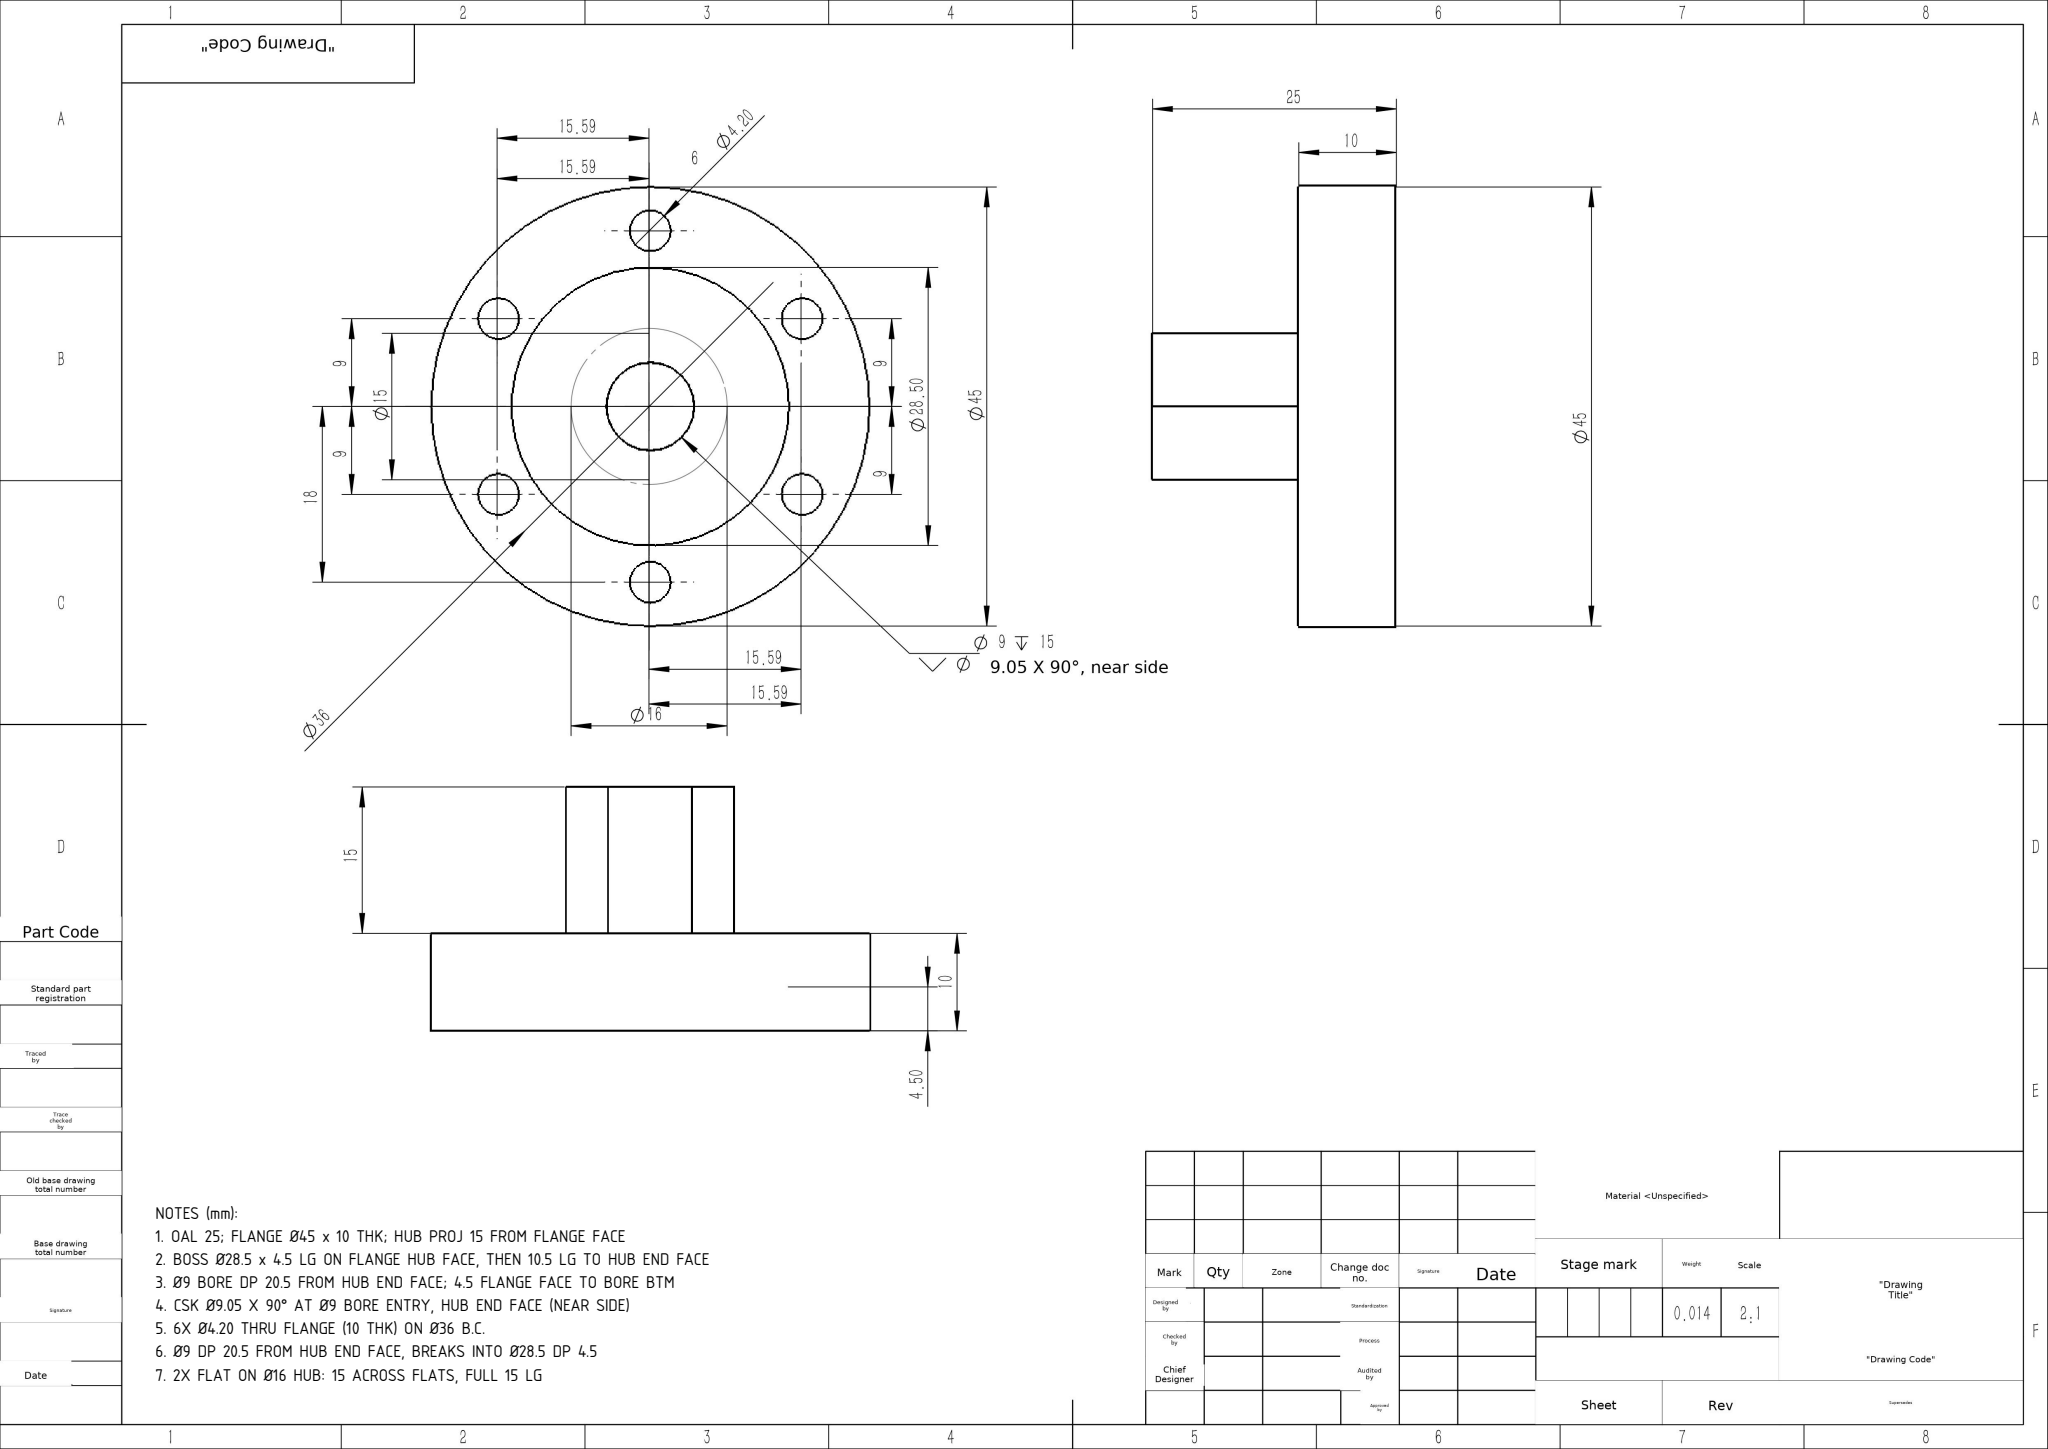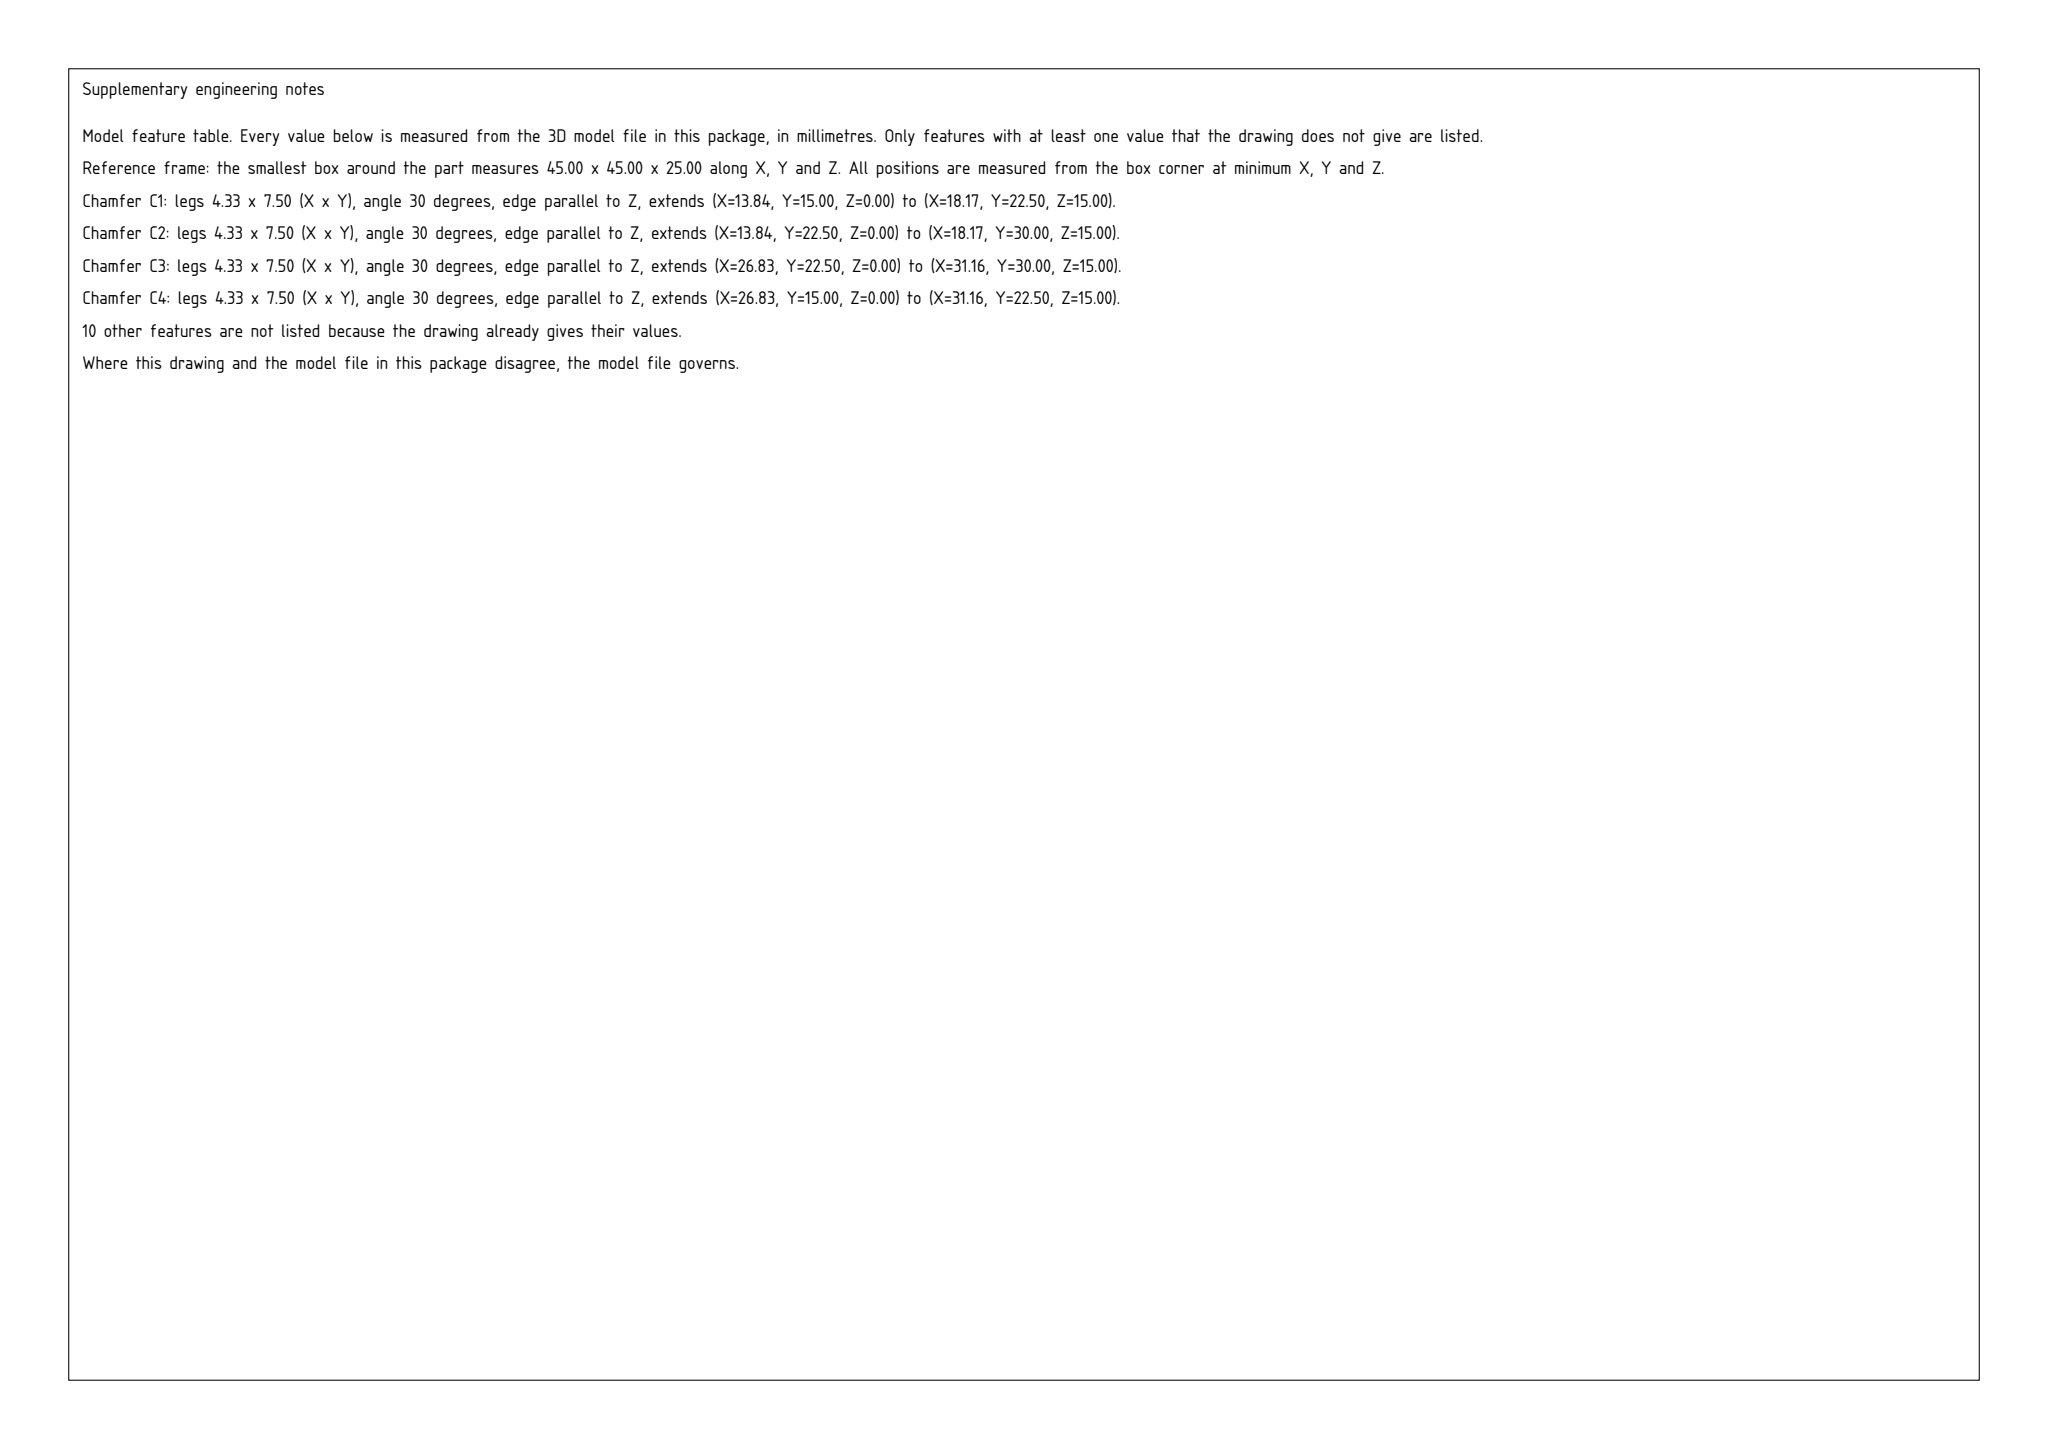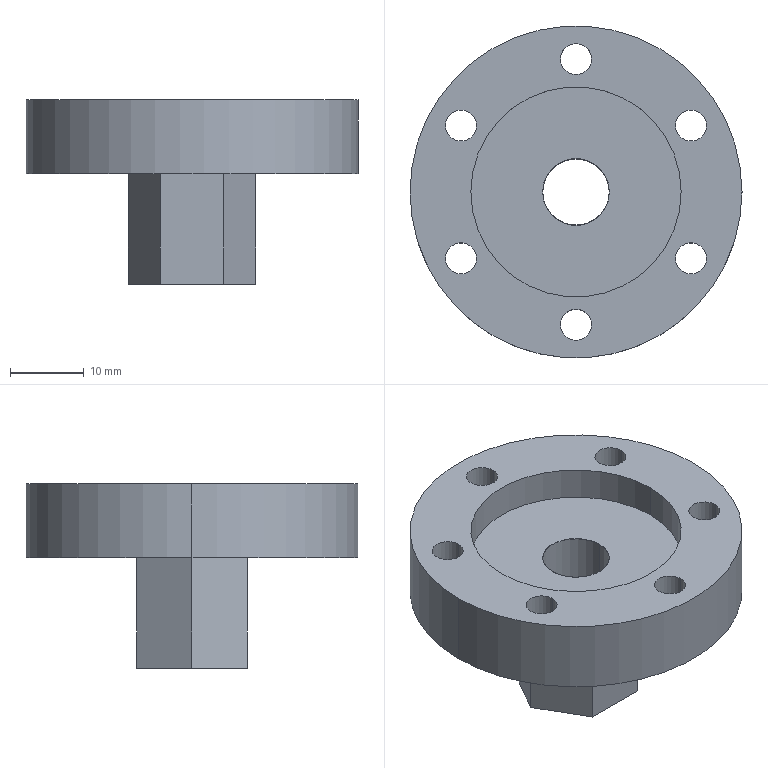Part | SolidWorks | mm | 1 solid | 30 faces | box 45 x 45 x 25 mm | volume 13821 mm3 | cylinder 18 | plane 10 | cone 2 | commonest cylinder face diameters 4.2 x12 9 x2 28.5 x2 45 x2
Drawing notes:
OAL 25; FLANGE Ø45 x 10 THK; HUB PROJ 15 FROM FLANGE FACE | from the solid: cyl Ø45 len 10; bbox z=25; z-planes 0,15,25 -> 25-10=15 hub
BOSS Ø28.5 x 4.5 LG ON FLANGE HUB FACE, THEN 10.5 LG TO HUB END FACE | from the solid: cyl [28.5,'z',(22.5,22.5),len 4.5] coaxial w/ Ø45; z-planes 0,15 -> 15-4.5=10.5
Ø9 BORE DP 20.5 FROM HUB END FACE; 4.5 FLANGE FACE TO BORE BTM | from the solid: cyl Ø9 len 20.48, z-plane 20.5; 25-20.5=4.5
CSK Ø9.05 X 90° AT Ø9 BORE ENTRY, HUB END FACE (NEAR SIDE) | from the solid: cones [90°, ref dia 9.05] at bore entry z=0
6X Ø4.20 THRU FLANGE (10 THK) ON Ø36 B.C. | from the solid: Six Ø4.2 z-axis cyls, length 10.0 = flange thickness (z15-25), centers at r=18 from axis (Ø36 B.C.)
Ø9 DP 20.5 FROM HUB END FACE, BREAKS INTO Ø28.5 DP 4.5 | from the solid: Ø9 cyl len 20.48 from z=0 to plane z=20.5; Ø28.5 cyl len 4.5 from z=20.5 to z=25 (flange back face)
2X FLAT ON Ø16 HUB: 15 ACROSS FLATS, FULL 15 LG | from the solid: Planes y=15.0 and y=30.0 (15 apart, symmetric about axis y=22.5) on hub z=0-15
build123d program:
from build123d import *

# Parameters (mm, degrees)
SKETCH1_R                               = 22.5
BOSS_EXTRUDE1_DEPTH                     = 10
SKETCH3_R                               = 14.25
CUT_EXTRUDE2_DEPTH                      = 4.5
SKETCH4_R                               = 2.1
CUT_EXTRUDE3_DEPTH                      = 34.354
M10X1_0_TAPPED_HOLE_DRILL_1_D           = 9
M10X1_0_TAPPED_HOLE_DRILL_1_DEPTH       = 15
M10X1_0_TAPPED_HOLE_DRILL_1_CSINK_D     = 9.05
M10X1_0_TAPPED_HOLE_DRILL_1_CSINK_ANGLE = 90
M10X1_0_TAPPED_HOLE_DRILL_1_TIP         = 2.704
BOSS_EXTRUDE2_START                     = 15
SKETCH8_R                               = 4.5
BOSS_EXTRUDE2_DEPTH                     = 15


with BuildPart() as part:
    # Sketch1 → Boss-Extrude1 (new body)
    with BuildSketch(Plane.XY):
        Circle(SKETCH1_R)
    extrude(amount=BOSS_EXTRUDE1_DEPTH)

    # Sketch3 → Cut-Extrude2 (cut)
    with BuildSketch(Plane.XY.offset(10)):
        Circle(SKETCH3_R)
    extrude(amount=-CUT_EXTRUDE2_DEPTH, mode=Mode.SUBTRACT)

    # Sketch4 → Cut-Extrude3 (cut, through all)
    with BuildSketch(Plane(origin=(0, 0, 0), x_dir=(-1, 0, 0), z_dir=(0, 0, -1))):
        with Locations((0, 18)):
            Circle(SKETCH4_R)
        with Locations((15.588, 9)):
            Circle(SKETCH4_R)
        with Locations((15.588, -9)):
            Circle(SKETCH4_R)
        with Locations((0, -18)):
            Circle(SKETCH4_R)
        with Locations((-15.588, -9)):
            Circle(SKETCH4_R)
        with Locations((-15.588, 9)):
            Circle(SKETCH4_R)
    extrude(amount=-CUT_EXTRUDE3_DEPTH, mode=Mode.SUBTRACT)

    # M10X1.0 Tapped Hole Drill 1
    with Locations(Plane.XY.offset(5.5)):
        with Locations((0, 0)):
            CounterSinkHole(M10X1_0_TAPPED_HOLE_DRILL_1_D / 2, M10X1_0_TAPPED_HOLE_DRILL_1_CSINK_D / 2, depth=M10X1_0_TAPPED_HOLE_DRILL_1_DEPTH, counter_sink_angle=M10X1_0_TAPPED_HOLE_DRILL_1_CSINK_ANGLE)
            with Locations((0, 0, -(M10X1_0_TAPPED_HOLE_DRILL_1_DEPTH + M10X1_0_TAPPED_HOLE_DRILL_1_TIP / 2))):  # 118° drill point
                Cone(0, M10X1_0_TAPPED_HOLE_DRILL_1_D / 2, M10X1_0_TAPPED_HOLE_DRILL_1_TIP, mode=Mode.SUBTRACT)

    # Sketch8 → Boss-Extrude2 (add)
    with BuildSketch(Plane(origin=(0, 0, 0), x_dir=(-1, 0, 0), z_dir=(0, 0, -1)).offset(BOSS_EXTRUDE2_START)):
        Polygon((8.66, 0), (4.33, 7.5), (-4.33, 7.5), (-8.66, 0), (-4.33, -7.5), (4.33, -7.5), align=None)
        with Locations(Location((0, 0, 0), (0, 0, 180))):
            Circle(SKETCH8_R, mode=Mode.SUBTRACT)
    extrude(amount=-BOSS_EXTRUDE2_DEPTH)


solid = part.part